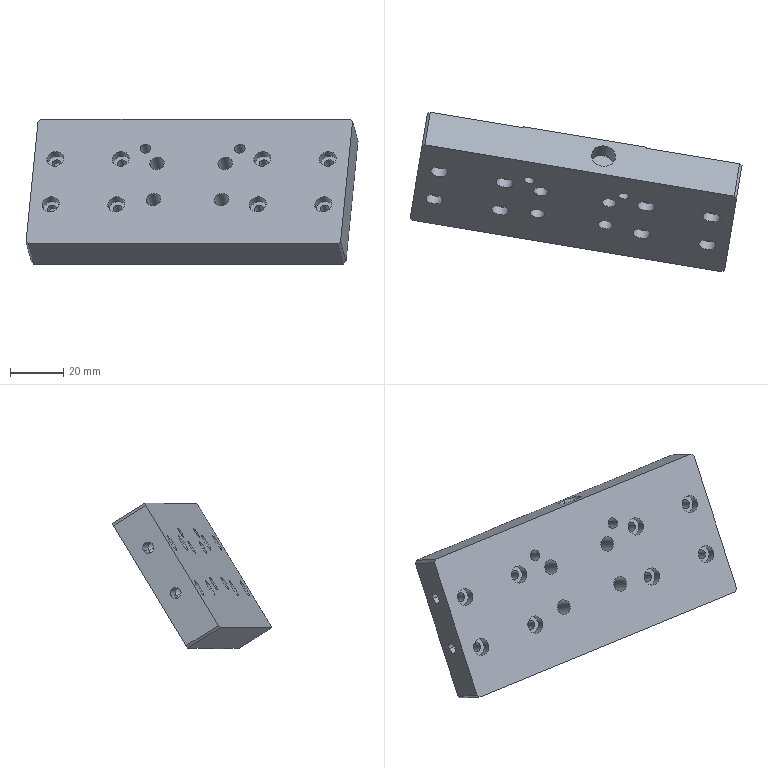Component | SolidWorks | 14AC-24-1-005-1 | 1 solid | 89 faces | box 124.95 x 59.91 x 54.74 mm | volume 91485 mm3 | cylinder 58 | plane 27 | cone 4 | commonest cylinder face diameters 6.5 x16 3.4 x16 10 x8 5.5 x8 4 x4 4.2 x4 9 x2
build123d program:
from build123d import *

# Parameters (mm, degrees)
SKETCH1_W                                       = 120
SKETCH1_H                                       = 55
BOSS_EXTRUDE1_DEPTH                             = 15
SKETCH3_W                                       = 40
SKETCH3_H                                       = 55
CUT_EXTRUDE2_DEPTH                              = 0.5
M3_HEX_SOCKET_HEAD_CAP_SCREW_CBORE1_D           = 3.4
M3_HEX_SOCKET_HEAD_CAP_SCREW_CBORE1_CBORE_D     = 6.5
M3_HEX_SOCKET_HEAD_CAP_SCREW_CBORE1_CBORE_DEPTH = 3.4
M5_HEX_SOCKET_HEAD_CAP_SCREW_CBORE1_D           = 5.5
M5_HEX_SOCKET_HEAD_CAP_SCREW_CBORE1_CBORE_D     = 10
M5_HEX_SOCKET_HEAD_CAP_SCREW_CBORE1_CBORE_DEPTH = 5.4
M5_TAPPED_HOLE3_D                               = 4.2
M5_TAPPED_HOLE3_DEPTH                           = 12.4
M5_TAPPED_HOLE3_TIP                             = 1.262
CHAMFER1_SIZE                                   = 1
SKETCH13_R                                      = 2
CUT_EXTRUDE3_DEPTH                              = 68.685
SKETCH14_R                                      = 4.5
CUT_EXTRUDE4_DEPTH                              = 7


with BuildPart() as part:
    # Sketch1 → Boss-Extrude1 (new body)
    with BuildSketch(Plane.XY):
        Rectangle(SKETCH1_W, SKETCH1_H)
    extrude(amount=BOSS_EXTRUDE1_DEPTH)

    # Sketch3 → Cut-Extrude2 (cut)
    with BuildSketch(Plane(origin=(0, 0, 0), x_dir=(-1, 0, 0), z_dir=(0, 0, -1))):
        with Locations((-43.5, 0)):
            Rectangle(SKETCH3_W, SKETCH3_H)
        with Locations((43.5, 0)):
            Rectangle(SKETCH3_W, SKETCH3_H)
    extrude(amount=-CUT_EXTRUDE2_DEPTH, mode=Mode.SUBTRACT)

    # M3 Hex Socket Head Cap Screw CBORE1 (through all)
    with Locations(Plane(origin=(27, 10, 15), x_dir=(1, 0, 0), z_dir=(0, 0, 1))):
        with Locations((0, 0), (25, 0), (0, -20), (25, -20)):
            m3_hex_socket_head_cap_screw_cbore1 = CounterBoreHole(M3_HEX_SOCKET_HEAD_CAP_SCREW_CBORE1_D / 2, M3_HEX_SOCKET_HEAD_CAP_SCREW_CBORE1_CBORE_D / 2, M3_HEX_SOCKET_HEAD_CAP_SCREW_CBORE1_CBORE_DEPTH)

    # Mirror1: M3 Hex Socket Head Cap Screw CBORE1 across plane
    add(m3_hex_socket_head_cap_screw_cbore1.mirror(Plane.ZY), mode=Mode.SUBTRACT)

    # M5 Hex Socket Head Cap Screw CBORE1 (through all)
    with Locations(Plane(origin=(13, 8, 0), x_dir=(-1, 0, 0), z_dir=(0, 0, -1))):
        with Locations((0, 0), (26, 0), (0, -16), (26, -16)):
            CounterBoreHole(M5_HEX_SOCKET_HEAD_CAP_SCREW_CBORE1_D / 2, M5_HEX_SOCKET_HEAD_CAP_SCREW_CBORE1_CBORE_D / 2, M5_HEX_SOCKET_HEAD_CAP_SCREW_CBORE1_CBORE_DEPTH)

    # M5 Tapped Hole3
    with Locations(Plane(origin=(-60, 12.5, 7.5), x_dir=(0, -1, 0), z_dir=(-1, 0, 0))):
        with Locations((0, 0), (20, 0)):
            Hole(M5_TAPPED_HOLE3_D / 2, depth=M5_TAPPED_HOLE3_DEPTH)
            with Locations((0, 0, -(M5_TAPPED_HOLE3_DEPTH + M5_TAPPED_HOLE3_TIP / 2))):  # 118° drill point
                Cone(0, M5_TAPPED_HOLE3_D / 2, M5_TAPPED_HOLE3_TIP, mode=Mode.SUBTRACT)

    # Chamfer1
    chamfer1_edges = [part.edges().sort_by_distance(p)[0] for p in [
        (60, -27.5, 7.75),
        (-60, -27.5, 7.75),
        (-60, 27.5, 7.75),
        (60, 27.5, 7.75),
    ]]
    chamfer(chamfer1_edges, length=CHAMFER1_SIZE)

    # Sketch13 → Cut-Extrude3 (cut, through all)
    with BuildSketch(Plane.XY.offset(15)):
        with Locations((18, 14.5)):
            Circle(SKETCH13_R)
        with Locations((-18, 14.5)):
            Circle(SKETCH13_R)
    extrude(amount=-CUT_EXTRUDE3_DEPTH, mode=Mode.SUBTRACT)

    # Sketch14 → Cut-Extrude4 (cut)
    with BuildSketch(Plane(origin=(0, 27.5, 0), x_dir=(1, 0, 0), z_dir=(0, 1, 0))):
        with Locations(Location((8, -7, 0), (0, 0, 270))):
            Circle(SKETCH14_R)
    extrude(amount=-CUT_EXTRUDE4_DEPTH, mode=Mode.SUBTRACT)


solid = part.part

# Placed as in the assembly
solid = solid.moved(Location((411.78, -139.664, -171.65), (58.173, -8.052, -4.969)))